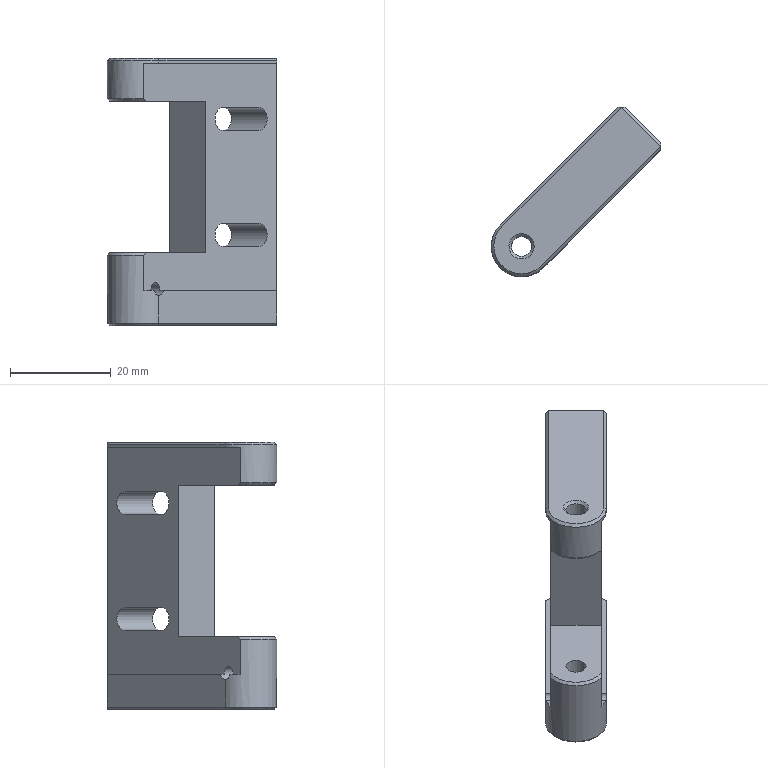Component | SolidWorks | UpperRollerAxisSeat-1 | 1 solid | 64 faces | volume 13628 mm3 | plane 32 | cylinder 18 | cone 14 | commonest cylinder face diameters 2.5 x4 4 x4 4.2 x4 4.6 x4 12 x2